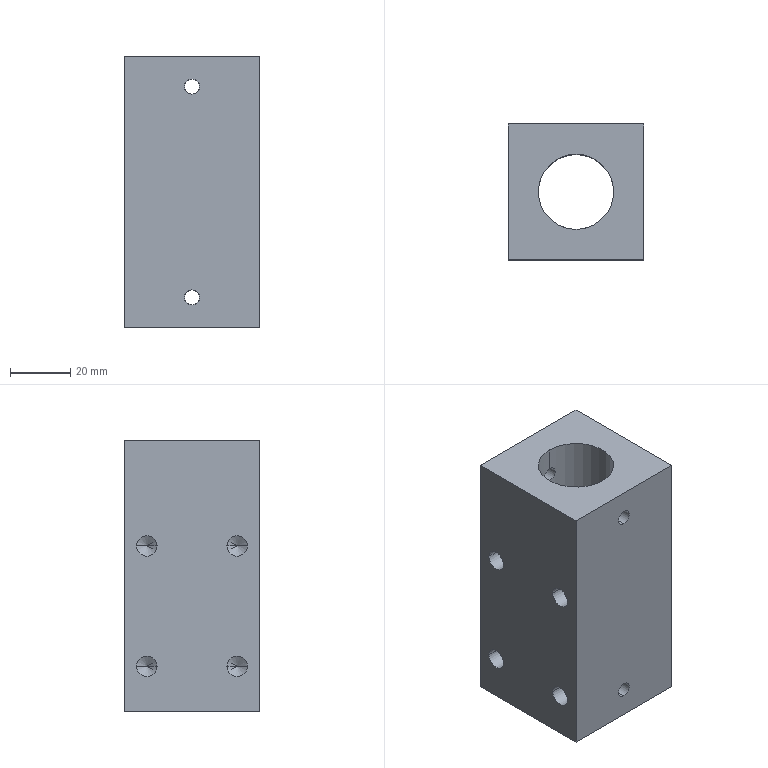Component | SolidWorks | LowerSideBeltXG-XG1-1_-LowerSleeveXG-XG1-1 | 1 solid | 48 faces | box 45 x 45 x 90 mm | volume 133016 mm3 | cylinder 26 | cone 16 | plane 6 | commonest cylinder face diameters 6.8 x16 5 x8 25 x2
build123d program:
from build123d import *

# Parameters (mm, degrees)
SKETCH1_W                  = 45
SKETCH1_H                  = 45
SKETCH1_R                  = 12.5
BOSS_EXTRUDE1_DEPTH        = 45
M8_TAPPED_HOLE1_AT_2_COUNT = 2
M8_TAPPED_HOLE1_AT_2_PITCH = 30
M8_TAPPED_HOLE1_AT_3_COUNT = 2
M8_TAPPED_HOLE1_AT_3_PITCH = 40
M8_TAPPED_HOLE1_AT_4_COUNT = 2
M8_TAPPED_HOLE1_AT_4_PITCH = 50
M6_TAPPED_HOLE1_D          = 5


with BuildPart() as part:
    # Sketch1 → Boss-Extrude1 (new, symmetric)
    with BuildSketch(Plane(origin=(0, 0, 0), x_dir=(0, 0, -1), z_dir=(1, 0, 0))):
        Rectangle(SKETCH1_W, SKETCH1_H)
        with Locations(Location((0, 0, 0), (0, 0, 180))):
            Circle(SKETCH1_R, mode=Mode.SUBTRACT)
    extrude(amount=BOSS_EXTRUDE1_DEPTH, both=True)

    # Sketch2 → M8 Tapped Hole1 (revolve, cut)
    with BuildSketch(Plane(origin=(-30, -22.5, 15), x_dir=(0, 0, -1), z_dir=(1, 0, 0))):
        Polygon((0, 0), (0, 16.043), (3.4, 14), (3.4, 0), align=None)
    m8_tapped_hole1 = revolve(axis=Axis((-30, -28.85, 15), (0, 1, 0)), mode=Mode.SUBTRACT)

    # M8 Tapped Hole1 at 2: M8 Tapped Hole1 ×2
    with Locations(*[(0, 0, -i * M8_TAPPED_HOLE1_AT_2_PITCH) for i in range(1, M8_TAPPED_HOLE1_AT_2_COUNT)]):
        add(m8_tapped_hole1, mode=Mode.SUBTRACT)

    # M8 Tapped Hole1 at 3: M8 Tapped Hole1 ×2
    with Locations(*[(i * M8_TAPPED_HOLE1_AT_3_PITCH, 0, 0) for i in range(1, M8_TAPPED_HOLE1_AT_3_COUNT)]):
        add(m8_tapped_hole1, mode=Mode.SUBTRACT)

    # M8 Tapped Hole1 at 4: M8 Tapped Hole1 ×2
    with Locations(*[Vector(0.8, 0, -0.6) * (i * M8_TAPPED_HOLE1_AT_4_PITCH) for i in range(1, M8_TAPPED_HOLE1_AT_4_COUNT)]):
        add(m8_tapped_hole1, mode=Mode.SUBTRACT)

    # Mirror1: M8 Tapped Hole1 across plane
    add(m8_tapped_hole1.mirror(Plane.ZX), mode=Mode.SUBTRACT)

    # Mirror1 copy 1 sketch → Mirror1 copy 1 (revolve, cut)
    with BuildSketch(Plane(origin=(-30, 22.5, -15), x_dir=(0, 0, -1), z_dir=(1, 0, 0))):
        Polygon((0, 0), (0, -16.043), (3.4, -14), (3.4, 0), align=None)
    revolve(axis=Axis((-30, 28.85, -15), (0, 1, 0)), mode=Mode.SUBTRACT)

    # Mirror1 copy 2 sketch → Mirror1 copy 2 (revolve, cut)
    with BuildSketch(Plane(origin=(10, 22.5, 15), x_dir=(0, 0, -1), z_dir=(1, 0, 0))):
        Polygon((0, 0), (0, -16.043), (3.4, -14), (3.4, 0), align=None)
    revolve(axis=Axis((10, 28.85, 15), (0, 1, 0)), mode=Mode.SUBTRACT)

    # Mirror1 copy 3 sketch → Mirror1 copy 3 (revolve, cut)
    with BuildSketch(Plane(origin=(10, 22.5, -15), x_dir=(0, 0, -1), z_dir=(1, 0, 0))):
        Polygon((0, 0), (0, -16.043), (3.4, -14), (3.4, 0), align=None)
    revolve(axis=Axis((10, 28.85, -15), (0, 1, 0)), mode=Mode.SUBTRACT)

    # M6 Tapped Hole1 (through all)
    with Locations(Plane.XY.offset(22.5)):
        with Locations((-35, 0), (35, 0)):
            Hole(M6_TAPPED_HOLE1_D / 2)


solid = part.part

# Placed as in the assembly
solid = solid.moved(Location((-348.72, 545, 114), (90, 0, 90)))